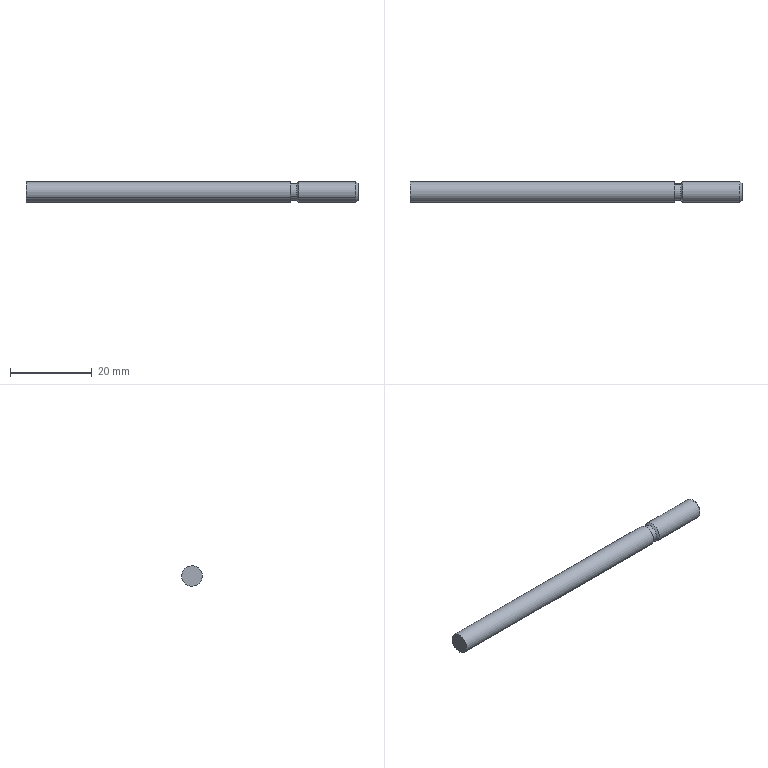Component | SolidWorks | A_CDJ2B16_60_B_0-1_CopyRod_A_CDJ2B16_60_B_0-1 | 1 solid | 13 faces | box 81 x 5 x 5 mm | volume 1576 mm3 | cylinder 6 | cone 4 | plane 3 | commonest cylinder face diameters 5 x4 4.02 x2
build123d program:
from build123d import *


with BuildPart() as part:
    # Sketch1 → Revolve1 (revolve)
    with BuildSketch(Plane(origin=(0, 0, 0), x_dir=(0, 0, -1), z_dir=(1, 0, 0)), mode=Mode.PRIVATE) as revolve1_sk:
        Polygon((-20, 0), (-20, 2.01), (-19.51, 2.5), (-5.49, 2.5), (-5, 2.01), (-3.5, 2.01), (-3.5, 2.5), (61, 2.5), (61, 0), align=None)
    revolve(revolve1_sk.sketch.rotate(Axis((0, 0, -61), (0, 0, 1)), 270), axis=Axis((0, 0, -61), (0, 0, 1)))


solid = part.part

# Placed as in the assembly
solid = solid.moved(Location((105.27, 22.768, 80.829), (0, 90, 0)))
STEP:
#1=COLOUR_RGB('',0.7922,0.8196,0.9333);
#2=FILL_AREA_STYLE_COLOUR('',#1);
#3=FILL_AREA_STYLE('',(#2));
#4=SURFACE_STYLE_FILL_AREA(#3);
#5=SURFACE_SIDE_STYLE('',(#4));
#6=SURFACE_STYLE_USAGE(.BOTH.,#5);
#7=PRESENTATION_STYLE_ASSIGNMENT((#6));
#8=CARTESIAN_POINT('',(1.743,0.8113,3.133));
#9=VERTEX_POINT('',#8);
#10=CARTESIAN_POINT('',(1.743,0.9815,3.232));
#11=VERTEX_POINT('',#10);
#12=CARTESIAN_POINT('',(1.743,0.8964,3.182));
#13=DIRECTION('',(1.,0.,0.));
#14=DIRECTION('',(0.,-0.8649,-0.502));
#15=AXIS2_PLACEMENT_3D('',#12,#13,#14);
#16=CIRCLE('',#15,0.09843);
#17=EDGE_CURVE('',#9,#11,#16,.T.);
#18=ORIENTED_EDGE('',*,*,#17,.T.);
#19=CARTESIAN_POINT('',(4.282,0.9815,3.232));
#20=VERTEX_POINT('',#19);
#21=CARTESIAN_POINT('',(1.743,0.9815,3.232));
#22=DIRECTION('',(1.,0.,0.));
#23=VECTOR('',#22,39.37);
#24=LINE('',#21,#23);
#25=EDGE_CURVE('',#11,#20,#24,.T.);
#26=ORIENTED_EDGE('',*,*,#25,.T.);
#27=CARTESIAN_POINT('',(4.282,0.8113,3.133));
#28=VERTEX_POINT('',#27);
#29=CARTESIAN_POINT('',(4.282,0.8964,3.182));
#30=DIRECTION('',(1.,0.,0.));
#31=DIRECTION('',(0.,-0.8649,-0.502));
#32=AXIS2_PLACEMENT_3D('',#29,#30,#31);
#33=CIRCLE('',#32,0.09843);
#34=EDGE_CURVE('',#28,#20,#33,.T.);
#35=ORIENTED_EDGE('',*,*,#34,.F.);
#36=CARTESIAN_POINT('',(1.743,0.8113,3.133));
#37=DIRECTION('',(1.,0.,0.));
#38=VECTOR('',#37,39.37);
#39=LINE('',#36,#38);
#40=EDGE_CURVE('',#9,#28,#39,.T.);
#41=ORIENTED_EDGE('',*,*,#40,.F.);
#42=EDGE_LOOP('',(#18,#26,#35,#41));
#43=FACE_OUTER_BOUND('',#42,.T.);
#44=CARTESIAN_POINT('',(1.743,0.8964,3.182));
#45=DIRECTION('',(1.,0.,0.));
#46=DIRECTION('',(0.,-0.8649,-0.502));
#47=AXIS2_PLACEMENT_3D('',#44,#45,#46);
#48=CYLINDRICAL_SURFACE('',#47,0.09843);
#49=ADVANCED_FACE('',(#43),#48,.T.);
#50=CARTESIAN_POINT('',(4.282,0.8279,3.143));
#51=VERTEX_POINT('',#50);
#52=CARTESIAN_POINT('',(4.282,0.9648,3.222));
#53=VERTEX_POINT('',#52);
#54=CARTESIAN_POINT('',(4.282,0.8964,3.182));
#55=DIRECTION('',(1.,0.,0.));
#56=DIRECTION('',(0.,-0.8649,-0.502));
#57=AXIS2_PLACEMENT_3D('',#54,#55,#56);
#58=CIRCLE('',#57,0.07913);
#59=EDGE_CURVE('',#51,#53,#58,.T.);
#60=ORIENTED_EDGE('',*,*,#59,.T.);
#61=CARTESIAN_POINT('',(4.341,0.9648,3.222));
#62=VERTEX_POINT('',#61);
#63=CARTESIAN_POINT('',(1.743,0.9648,3.222));
#64=DIRECTION('',(1.,0.,0.));
#65=VECTOR('',#64,39.37);
#66=LINE('',#63,#65);
#67=EDGE_CURVE('',#53,#62,#66,.T.);
#68=ORIENTED_EDGE('',*,*,#67,.T.);
#69=CARTESIAN_POINT('',(4.341,0.8279,3.143));
#70=VERTEX_POINT('',#69);
#71=CARTESIAN_POINT('',(4.341,0.8964,3.182));
#72=DIRECTION('',(1.,0.,0.));
#73=DIRECTION('',(0.,-0.8649,-0.502));
#74=AXIS2_PLACEMENT_3D('',#71,#72,#73);
#75=CIRCLE('',#74,0.07913);
#76=EDGE_CURVE('',#70,#62,#75,.T.);
#77=ORIENTED_EDGE('',*,*,#76,.F.);
#78=CARTESIAN_POINT('',(1.743,0.8279,3.143));
#79=DIRECTION('',(1.,0.,0.));
#80=VECTOR('',#79,39.37);
#81=LINE('',#78,#80);
#82=EDGE_CURVE('',#51,#70,#81,.T.);
#83=ORIENTED_EDGE('',*,*,#82,.F.);
#84=EDGE_LOOP('',(#60,#68,#77,#83));
#85=FACE_OUTER_BOUND('',#84,.T.);
#86=CARTESIAN_POINT('',(1.743,0.8964,3.182));
#87=DIRECTION('',(1.,0.,0.));
#88=DIRECTION('',(0.,-0.8649,-0.502));
#89=AXIS2_PLACEMENT_3D('',#86,#87,#88);
#90=CYLINDRICAL_SURFACE('',#89,0.07913);
#91=ADVANCED_FACE('',(#85),#90,.T.);
#92=ORIENTED_EDGE('',*,*,#76,.T.);
#93=CARTESIAN_POINT('',(4.361,0.9815,3.232));
#94=VERTEX_POINT('',#93);
#95=CARTESIAN_POINT('',(4.341,0.9648,3.222));
#96=DIRECTION('',(0.7071,0.6116,0.3549));
#97=VECTOR('',#96,39.37);
#98=LINE('',#95,#97);
#99=EDGE_CURVE('',#62,#94,#98,.T.);
#100=ORIENTED_EDGE('',*,*,#99,.T.);
#101=CARTESIAN_POINT('',(4.361,0.8113,3.133));
#102=VERTEX_POINT('',#101);
#103=CARTESIAN_POINT('',(4.361,0.8964,3.182));
#104=DIRECTION('',(1.,0.,0.));
#105=DIRECTION('',(0.,-0.8649,-0.502));
#106=AXIS2_PLACEMENT_3D('',#103,#104,#105);
#107=CIRCLE('',#106,0.09843);
#108=EDGE_CURVE('',#102,#94,#107,.T.);
#109=ORIENTED_EDGE('',*,*,#108,.F.);
#110=CARTESIAN_POINT('',(4.341,0.8279,3.143));
#111=DIRECTION('',(0.7071,-0.6116,-0.3549));
#112=VECTOR('',#111,39.37);
#113=LINE('',#110,#112);
#114=EDGE_CURVE('',#70,#102,#113,.T.);
#115=ORIENTED_EDGE('',*,*,#114,.F.);
#116=EDGE_LOOP('',(#92,#100,#109,#115));
#117=FACE_OUTER_BOUND('',#116,.T.);
#118=CARTESIAN_POINT('',(4.341,0.8964,3.182));
#119=DIRECTION('',(1.,0.,0.));
#120=DIRECTION('',(0.,-0.8649,-0.502));
#121=AXIS2_PLACEMENT_3D('',#118,#119,#120);
#122=CONICAL_SURFACE('',#121,0.07913,0.7854);
#123=ADVANCED_FACE('',(#117),#122,.T.);
#124=ORIENTED_EDGE('',*,*,#108,.T.);
#125=CARTESIAN_POINT('',(4.913,0.9815,3.232));
#126=VERTEX_POINT('',#125);
#127=CARTESIAN_POINT('',(1.743,0.9815,3.232));
#128=DIRECTION('',(1.,0.,0.));
#129=VECTOR('',#128,39.37);
#130=LINE('',#127,#129);
#131=EDGE_CURVE('',#94,#126,#130,.T.);
#132=ORIENTED_EDGE('',*,*,#131,.T.);
#133=CARTESIAN_POINT('',(4.913,0.8113,3.133));
#134=VERTEX_POINT('',#133);
#135=CARTESIAN_POINT('',(4.913,0.8964,3.182));
#136=DIRECTION('',(1.,0.,0.));
#137=DIRECTION('',(0.,-0.8649,-0.502));
#138=AXIS2_PLACEMENT_3D('',#135,#136,#137);
#139=CIRCLE('',#138,0.09843);
#140=EDGE_CURVE('',#134,#126,#139,.T.);
#141=ORIENTED_EDGE('',*,*,#140,.F.);
#142=CARTESIAN_POINT('',(1.743,0.8113,3.133));
#143=DIRECTION('',(1.,0.,0.));
#144=VECTOR('',#143,39.37);
#145=LINE('',#142,#144);
#146=EDGE_CURVE('',#102,#134,#145,.T.);
#147=ORIENTED_EDGE('',*,*,#146,.F.);
#148=EDGE_LOOP('',(#124,#132,#141,#147));
#149=FACE_OUTER_BOUND('',#148,.T.);
#150=CARTESIAN_POINT('',(1.743,0.8964,3.182));
#151=DIRECTION('',(1.,0.,0.));
#152=DIRECTION('',(0.,-0.8649,-0.502));
#153=AXIS2_PLACEMENT_3D('',#150,#151,#152);
#154=CYLINDRICAL_SURFACE('',#153,0.09843);
#155=ADVANCED_FACE('',(#149),#154,.T.);
#156=CARTESIAN_POINT('',(4.932,0.8279,3.143));
#157=VERTEX_POINT('',#156);
#158=CARTESIAN_POINT('',(4.932,0.9648,3.222));
#159=VERTEX_POINT('',#158);
#160=CARTESIAN_POINT('',(4.932,0.8964,3.182));
#161=DIRECTION('',(1.,0.,0.));
#162=DIRECTION('',(0.,-0.8649,-0.502));
#163=AXIS2_PLACEMENT_3D('',#160,#161,#162);
#164=CIRCLE('',#163,0.07913);
#165=EDGE_CURVE('',#157,#159,#164,.T.);
#166=ORIENTED_EDGE('',*,*,#165,.F.);
#167=CARTESIAN_POINT('',(4.913,0.8113,3.133));
#168=DIRECTION('',(-0.7071,-0.6116,-0.3549));
#169=VECTOR('',#168,39.37);
#170=LINE('',#167,#169);
#171=EDGE_CURVE('',#157,#134,#170,.T.);
#172=ORIENTED_EDGE('',*,*,#171,.T.);
#173=ORIENTED_EDGE('',*,*,#140,.T.);
#174=CARTESIAN_POINT('',(4.913,0.9815,3.232));
#175=DIRECTION('',(-0.7071,0.6116,0.3549));
#176=VECTOR('',#175,39.37);
#177=LINE('',#174,#176);
#178=EDGE_CURVE('',#159,#126,#177,.T.);
#179=ORIENTED_EDGE('',*,*,#178,.F.);
#180=EDGE_LOOP('',(#166,#172,#173,#179));
#181=FACE_OUTER_BOUND('',#180,.T.);
#182=CARTESIAN_POINT('',(4.913,0.8964,3.182));
#183=DIRECTION('',(-1.,-0.,-0.));
#184=DIRECTION('',(0.,0.8649,0.502));
#185=AXIS2_PLACEMENT_3D('',#182,#183,#184);
#186=CONICAL_SURFACE('',#185,0.09843,0.7854);
#187=ADVANCED_FACE('',(#181),#186,.T.);
#188=CARTESIAN_POINT('',(4.932,0.8964,3.182));
#189=DIRECTION('',(1.,0.,0.));
#190=DIRECTION('',(0.,-0.8649,-0.502));
#191=AXIS2_PLACEMENT_3D('',#188,#189,#190);
#192=CIRCLE('',#191,0.07913);
#193=EDGE_CURVE('',#159,#157,#192,.T.);
#194=ORIENTED_EDGE('',*,*,#193,.T.);
#195=ORIENTED_EDGE('',*,*,#165,.T.);
#196=EDGE_LOOP('',(#194,#195));
#197=FACE_OUTER_BOUND('',#196,.T.);
#198=CARTESIAN_POINT('',(4.932,0.8964,3.182));
#199=DIRECTION('',(-1.,-0.,-0.));
#200=DIRECTION('',(-0.,0.8649,0.502));
#201=AXIS2_PLACEMENT_3D('',#198,#199,#200);
#202=PLANE('',#201);
#203=ADVANCED_FACE('',(#197),#202,.F.);
#204=ORIENTED_EDGE('',*,*,#171,.F.);
#205=ORIENTED_EDGE('',*,*,#193,.F.);
#206=ORIENTED_EDGE('',*,*,#178,.T.);
#207=CARTESIAN_POINT('',(4.913,0.8964,3.182));
#208=DIRECTION('',(1.,0.,0.));
#209=DIRECTION('',(0.,-0.8649,-0.502));
#210=AXIS2_PLACEMENT_3D('',#207,#208,#209);
#211=CIRCLE('',#210,0.09843);
#212=EDGE_CURVE('',#126,#134,#211,.T.);
#213=ORIENTED_EDGE('',*,*,#212,.T.);
#214=EDGE_LOOP('',(#204,#205,#206,#213));
#215=FACE_OUTER_BOUND('',#214,.T.);
#216=CARTESIAN_POINT('',(4.913,0.8964,3.182));
#217=DIRECTION('',(-1.,-0.,-0.));
#218=DIRECTION('',(0.,0.8649,0.502));
#219=AXIS2_PLACEMENT_3D('',#216,#217,#218);
#220=CONICAL_SURFACE('',#219,0.09843,0.7854);
#221=ADVANCED_FACE('',(#215),#220,.T.);
#222=ORIENTED_EDGE('',*,*,#131,.F.);
#223=CARTESIAN_POINT('',(4.361,0.8964,3.182));
#224=DIRECTION('',(1.,0.,0.));
#225=DIRECTION('',(0.,-0.8649,-0.502));
#226=AXIS2_PLACEMENT_3D('',#223,#224,#225);
#227=CIRCLE('',#226,0.09843);
#228=EDGE_CURVE('',#94,#102,#227,.T.);
#229=ORIENTED_EDGE('',*,*,#228,.T.);
#230=ORIENTED_EDGE('',*,*,#146,.T.);
#231=ORIENTED_EDGE('',*,*,#212,.F.);
#232=EDGE_LOOP('',(#222,#229,#230,#231));
#233=FACE_OUTER_BOUND('',#232,.T.);
#234=CARTESIAN_POINT('',(1.743,0.8964,3.182));
#235=DIRECTION('',(1.,0.,0.));
#236=DIRECTION('',(0.,-0.8649,-0.502));
#237=AXIS2_PLACEMENT_3D('',#234,#235,#236);
#238=CYLINDRICAL_SURFACE('',#237,0.09843);
#239=ADVANCED_FACE('',(#233),#238,.T.);
#240=ORIENTED_EDGE('',*,*,#99,.F.);
#241=CARTESIAN_POINT('',(4.341,0.8964,3.182));
#242=DIRECTION('',(1.,0.,0.));
#243=DIRECTION('',(0.,-0.8649,-0.502));
#244=AXIS2_PLACEMENT_3D('',#241,#242,#243);
#245=CIRCLE('',#244,0.07913);
#246=EDGE_CURVE('',#62,#70,#245,.T.);
#247=ORIENTED_EDGE('',*,*,#246,.T.);
#248=ORIENTED_EDGE('',*,*,#114,.T.);
#249=ORIENTED_EDGE('',*,*,#228,.F.);
#250=EDGE_LOOP('',(#240,#247,#248,#249));
#251=FACE_OUTER_BOUND('',#250,.T.);
#252=CARTESIAN_POINT('',(4.341,0.8964,3.182));
#253=DIRECTION('',(1.,0.,0.));
#254=DIRECTION('',(0.,-0.8649,-0.502));
#255=AXIS2_PLACEMENT_3D('',#252,#253,#254);
#256=CONICAL_SURFACE('',#255,0.07913,0.7854);
#257=ADVANCED_FACE('',(#251),#256,.T.);
#258=ORIENTED_EDGE('',*,*,#67,.F.);
#259=CARTESIAN_POINT('',(4.282,0.8964,3.182));
#260=DIRECTION('',(1.,0.,0.));
#261=DIRECTION('',(0.,-0.8649,-0.502));
#262=AXIS2_PLACEMENT_3D('',#259,#260,#261);
#263=CIRCLE('',#262,0.07913);
#264=EDGE_CURVE('',#53,#51,#263,.T.);
#265=ORIENTED_EDGE('',*,*,#264,.T.);
#266=ORIENTED_EDGE('',*,*,#82,.T.);
#267=ORIENTED_EDGE('',*,*,#246,.F.);
#268=EDGE_LOOP('',(#258,#265,#266,#267));
#269=FACE_OUTER_BOUND('',#268,.T.);
#270=CARTESIAN_POINT('',(1.743,0.8964,3.182));
#271=DIRECTION('',(1.,0.,0.));
#272=DIRECTION('',(0.,-0.8649,-0.502));
#273=AXIS2_PLACEMENT_3D('',#270,#271,#272);
#274=CYLINDRICAL_SURFACE('',#273,0.07913);
#275=ADVANCED_FACE('',(#269),#274,.T.);
#276=ORIENTED_EDGE('',*,*,#59,.F.);
#277=ORIENTED_EDGE('',*,*,#264,.F.);
#278=EDGE_LOOP('',(#276,#277));
#279=FACE_BOUND('',#278,.T.);
#280=ORIENTED_EDGE('',*,*,#34,.T.);
#281=CARTESIAN_POINT('',(4.282,0.8964,3.182));
#282=DIRECTION('',(1.,0.,0.));
#283=DIRECTION('',(0.,-0.8649,-0.502));
#284=AXIS2_PLACEMENT_3D('',#281,#282,#283);
#285=CIRCLE('',#284,0.09843);
#286=EDGE_CURVE('',#20,#28,#285,.T.);
#287=ORIENTED_EDGE('',*,*,#286,.T.);
#288=EDGE_LOOP('',(#280,#287));
#289=FACE_OUTER_BOUND('',#288,.T.);
#290=CARTESIAN_POINT('',(4.282,0.9361,3.114));
#291=DIRECTION('',(-1.,-0.,-0.));
#292=DIRECTION('',(-0.,0.8649,0.502));
#293=AXIS2_PLACEMENT_3D('',#290,#291,#292);
#294=PLANE('',#293);
#295=ADVANCED_FACE('',(#279,#289),#294,.F.);
#296=ORIENTED_EDGE('',*,*,#25,.F.);
#297=CARTESIAN_POINT('',(1.743,0.8964,3.182));
#298=DIRECTION('',(1.,0.,0.));
#299=DIRECTION('',(0.,-0.8649,-0.502));
#300=AXIS2_PLACEMENT_3D('',#297,#298,#299);
#301=CIRCLE('',#300,0.09843);
#302=EDGE_CURVE('',#11,#9,#301,.T.);
#303=ORIENTED_EDGE('',*,*,#302,.T.);
#304=ORIENTED_EDGE('',*,*,#40,.T.);
#305=ORIENTED_EDGE('',*,*,#286,.F.);
#306=EDGE_LOOP('',(#296,#303,#304,#305));
#307=FACE_OUTER_BOUND('',#306,.T.);
#308=CARTESIAN_POINT('',(1.743,0.8964,3.182));
#309=DIRECTION('',(1.,0.,0.));
#310=DIRECTION('',(0.,-0.8649,-0.502));
#311=AXIS2_PLACEMENT_3D('',#308,#309,#310);
#312=CYLINDRICAL_SURFACE('',#311,0.09843);
#313=ADVANCED_FACE('',(#307),#312,.T.);
#314=ORIENTED_EDGE('',*,*,#17,.F.);
#315=ORIENTED_EDGE('',*,*,#302,.F.);
#316=EDGE_LOOP('',(#314,#315));
#317=FACE_OUTER_BOUND('',#316,.T.);
#318=CARTESIAN_POINT('',(1.743,0.9458,3.097));
#319=DIRECTION('',(1.,0.,0.));
#320=DIRECTION('',(0.,-0.8649,-0.502));
#321=AXIS2_PLACEMENT_3D('',#318,#319,#320);
#322=PLANE('',#321);
#323=ADVANCED_FACE('',(#317),#322,.F.);
#324=CLOSED_SHELL('',(#49,#91,#123,#155,#187,#203,#221,#239,#257,#275,#295,#313,#323));
#325=MANIFOLD_SOLID_BREP('',#324);
#326=STYLED_ITEM('',(#7),#325);
#327=PRESENTATION_LAYER_ASSIGNMENT('','',(#326));
#328=CARTESIAN_POINT('',(0.,0.,0.));
#329=DIRECTION('',(0.,0.,1.));
#330=DIRECTION('',(1.,0.,0.));
#331=AXIS2_PLACEMENT_3D('',#328,#329,#330);
#332=(LENGTH_UNIT()NAMED_UNIT(*)SI_UNIT($,.METRE.));
#333=LENGTH_MEASURE_WITH_UNIT(LENGTH_MEASURE(0.0254),#332);
#334=DIMENSIONAL_EXPONENTS(1.,0.,0.,0.,0.,0.,0.);
#335=(CONVERSION_BASED_UNIT('',#333)LENGTH_UNIT()NAMED_UNIT(#334));
#336=UNCERTAINTY_MEASURE_WITH_UNIT(LENGTH_MEASURE(0.00001),#335,'','');
#337=(NAMED_UNIT(*)PLANE_ANGLE_UNIT()SI_UNIT($,.RADIAN.));
#338=(NAMED_UNIT(*)SI_UNIT($,.STERADIAN.)SOLID_ANGLE_UNIT());
#339=(GEOMETRIC_REPRESENTATION_CONTEXT(3)GLOBAL_UNCERTAINTY_ASSIGNED_CONTEXT((#336))GLOBAL_UNIT_ASSIGNED_CONTEXT((#335,#337,#338))REPRESENTATION_CONTEXT('',''));
#340=ADVANCED_BREP_SHAPE_REPRESENTATION('',(#325,#331),#339);
#341=(LENGTH_UNIT()NAMED_UNIT(*)SI_UNIT($,.METRE.));
#342=LENGTH_MEASURE_WITH_UNIT(LENGTH_MEASURE(0.0254),#341);
#343=DIMENSIONAL_EXPONENTS(1.,0.,0.,0.,0.,0.,0.);
#344=(CONVERSION_BASED_UNIT('',#342)LENGTH_UNIT()NAMED_UNIT(#343));
#345=UNCERTAINTY_MEASURE_WITH_UNIT(LENGTH_MEASURE(0.00001),#344,'','');
#346=(NAMED_UNIT(*)PLANE_ANGLE_UNIT()SI_UNIT($,.RADIAN.));
#347=(NAMED_UNIT(*)SI_UNIT($,.STERADIAN.)SOLID_ANGLE_UNIT());
#348=(GEOMETRIC_REPRESENTATION_CONTEXT(3)GLOBAL_UNCERTAINTY_ASSIGNED_CONTEXT((#345))GLOBAL_UNIT_ASSIGNED_CONTEXT((#344,#346,#347))REPRESENTATION_CONTEXT('',''));
#349=MECHANICAL_DESIGN_GEOMETRIC_PRESENTATION_REPRESENTATION('',(#326),#348);